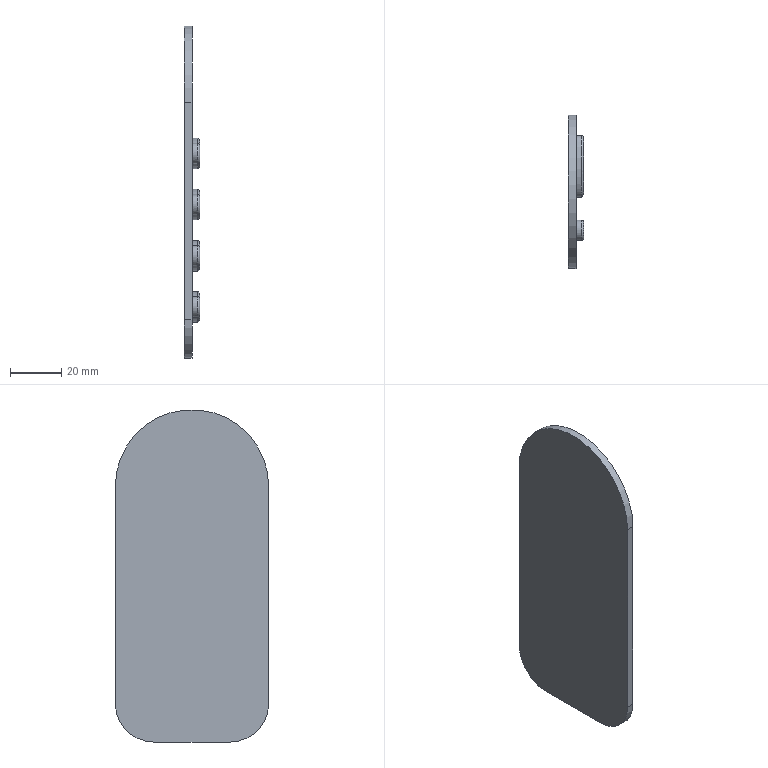Component | NX | CONTROL_PANEL | 9 solids | 40 faces | volume 25194 mm3 | plane 21 | cylinder 7 | other 4 | spline 4 | torus 4 | commonest cylinder face diameters 8 x4 30 x2 60 x1